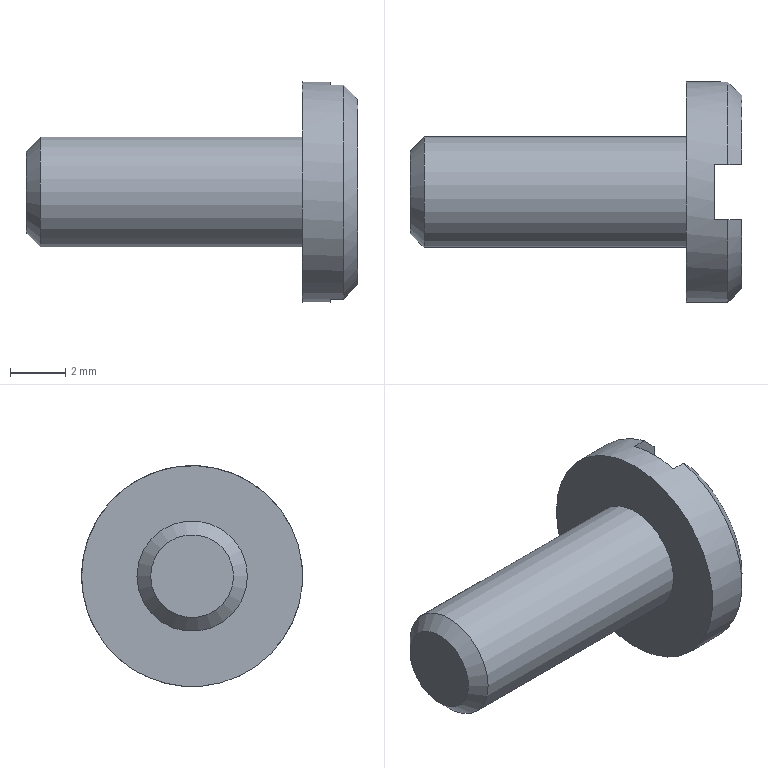Component | NX | SCREW | 1 solid | 12 faces | box 12 x 8 x 8 mm | volume 206 mm3 | plane 7 | cone 3 | cylinder 2 | commonest cylinder face diameters 4 x1 8 x1
STEP:
#1=CARTESIAN_POINT('',(0.,0.,0.));
#2=DIRECTION('',(0.,0.,1.));
#3=DIRECTION('',(1.,0.,0.));
#4=AXIS2_PLACEMENT_3D('',#1,#2,#3);
#5=CARTESIAN_POINT('',(63.511,118.396,33.354));
#6=VERTEX_POINT('',#5);
#7=CARTESIAN_POINT('',(63.511,118.396,26.646));
#8=VERTEX_POINT('',#7);
#9=CARTESIAN_POINT('',(63.511,118.396,35.5));
#10=DIRECTION('',(0.,0.,-1.));
#11=VECTOR('',#10,1.);
#12=LINE('',#9,#11);
#13=CARTESIAN_POINT('',(63.511,119.396,30.));
#14=DIRECTION('',(1.,0.,0.));
#15=DIRECTION('',(0.,1.,0.));
#16=AXIS2_PLACEMENT_3D('',#13,#14,#15);
#17=PLANE('',#16);
#18=CARTESIAN_POINT('',(-1.,5.5));
#19=DIRECTION('',(0.,-1.));
#20=VECTOR('',#19,1.);
#21=LINE('',#18,#20);
#22=(GEOMETRIC_REPRESENTATION_CONTEXT(2)PARAMETRIC_REPRESENTATION_CONTEXT()REPRESENTATION_CONTEXT('',''));
#23=DEFINITIONAL_REPRESENTATION('',(#21),#22);
#24=PCURVE('',#17,#23);
#25=CARTESIAN_POINT('',(62.511,118.396,35.5));
#26=DIRECTION('',(0.,-1.,-0.));
#27=DIRECTION('',(0.,0.,-1.));
#28=AXIS2_PLACEMENT_3D('',#25,#26,#27);
#29=PLANE('',#28);
#30=CARTESIAN_POINT('',(0.,1.));
#31=DIRECTION('',(1.,0.));
#32=VECTOR('',#31,1.);
#33=LINE('',#30,#32);
#34=(GEOMETRIC_REPRESENTATION_CONTEXT(2)PARAMETRIC_REPRESENTATION_CONTEXT()REPRESENTATION_CONTEXT('',''));
#35=DEFINITIONAL_REPRESENTATION('',(#33),#34);
#36=PCURVE('',#29,#35);
#37=SURFACE_CURVE('',#12,(#24,#36),.PCURVE_S1.);
#38=EDGE_CURVE('',#6,#8,#37,.T.);
#39=ORIENTED_EDGE('',*,*,#38,.F.);
#40=CARTESIAN_POINT('',(63.511,119.396,30.));
#41=DIRECTION('',(1.,0.,0.));
#42=DIRECTION('',(0.,1.,0.));
#43=AXIS2_PLACEMENT_3D('',#40,#41,#42);
#44=CIRCLE('',#43,3.5);
#45=CARTESIAN_POINT('',(0.,0.));
#46=DIRECTION('',(1.,0.));
#47=AXIS2_PLACEMENT_2D('',#45,#46);
#48=CIRCLE('',#47,3.5);
#49=(GEOMETRIC_REPRESENTATION_CONTEXT(2)PARAMETRIC_REPRESENTATION_CONTEXT()REPRESENTATION_CONTEXT('',''));
#50=DEFINITIONAL_REPRESENTATION('',(#48),#49);
#51=PCURVE('',#17,#50);
#52=CARTESIAN_POINT('',(63.511,119.396,30.));
#53=DIRECTION('',(-1.,0.,0.));
#54=DIRECTION('',(0.,-1.,0.));
#55=AXIS2_PLACEMENT_3D('',#52,#53,#54);
#56=CONICAL_SURFACE('',#55,3.5,0.7854);
#57=CARTESIAN_POINT('',(9.425,0.));
#58=DIRECTION('',(-1.,0.));
#59=VECTOR('',#58,1.);
#60=LINE('',#57,#59);
#61=(GEOMETRIC_REPRESENTATION_CONTEXT(2)PARAMETRIC_REPRESENTATION_CONTEXT()REPRESENTATION_CONTEXT('',''));
#62=DEFINITIONAL_REPRESENTATION('',(#60),#61);
#63=PCURVE('',#56,#62);
#64=SURFACE_CURVE('',#44,(#51,#63),.PCURVE_S1.);
#65=EDGE_CURVE('',#6,#8,#64,.T.);
#66=ORIENTED_EDGE('',*,*,#65,.T.);
#67=EDGE_LOOP('',(#39,#66));
#68=FACE_BOUND('',#67,.T.);
#69=ADVANCED_FACE('',(#68),#17,.T.);
#70=CARTESIAN_POINT('',(52.011,121.396,30.));
#71=VERTEX_POINT('',#70);
#72=CARTESIAN_POINT('',(52.011,119.396,30.));
#73=DIRECTION('',(1.,0.,0.));
#74=DIRECTION('',(0.,1.,0.));
#75=AXIS2_PLACEMENT_3D('',#72,#73,#74);
#76=CIRCLE('',#75,2.);
#77=CARTESIAN_POINT('',(61.511,119.396,30.));
#78=DIRECTION('',(-1.,0.,0.));
#79=DIRECTION('',(0.,-1.,0.));
#80=AXIS2_PLACEMENT_3D('',#77,#78,#79);
#81=CYLINDRICAL_SURFACE('',#80,2.);
#82=CARTESIAN_POINT('',(9.425,9.5));
#83=DIRECTION('',(-1.,0.));
#84=VECTOR('',#83,1.);
#85=LINE('',#82,#84);
#86=(GEOMETRIC_REPRESENTATION_CONTEXT(2)PARAMETRIC_REPRESENTATION_CONTEXT()REPRESENTATION_CONTEXT('',''));
#87=DEFINITIONAL_REPRESENTATION('',(#85),#86);
#88=PCURVE('',#81,#87);
#89=CARTESIAN_POINT('',(52.011,119.396,30.));
#90=DIRECTION('',(1.,0.,0.));
#91=DIRECTION('',(0.,1.,0.));
#92=AXIS2_PLACEMENT_3D('',#89,#90,#91);
#93=CONICAL_SURFACE('',#92,2.,0.7854);
#94=CARTESIAN_POINT('',(0.,0.));
#95=DIRECTION('',(1.,0.));
#96=VECTOR('',#95,1.);
#97=LINE('',#94,#96);
#98=(GEOMETRIC_REPRESENTATION_CONTEXT(2)PARAMETRIC_REPRESENTATION_CONTEXT()REPRESENTATION_CONTEXT('',''));
#99=DEFINITIONAL_REPRESENTATION('',(#97),#98);
#100=PCURVE('',#93,#99);
#101=SURFACE_CURVE('',#76,(#88,#100),.PCURVE_S1.);
#102=EDGE_CURVE('',#71,#71,#101,.T.);
#103=ORIENTED_EDGE('',*,*,#102,.T.);
#104=CARTESIAN_POINT('',(61.511,121.396,30.));
#105=VERTEX_POINT('',#104);
#106=CARTESIAN_POINT('',(61.511,121.396,30.));
#107=CARTESIAN_POINT('',(52.011,121.396,30.));
#108=B_SPLINE_CURVE_WITH_KNOTS('',1,(#106,#107),.UNSPECIFIED.,.F.,.F.,(2,2),(0.,9.5),.PIECEWISE_BEZIER_KNOTS.);
#109=CARTESIAN_POINT('',(3.142,0.));
#110=DIRECTION('',(0.,1.));
#111=VECTOR('',#110,1.);
#112=LINE('',#109,#111);
#113=(GEOMETRIC_REPRESENTATION_CONTEXT(2)PARAMETRIC_REPRESENTATION_CONTEXT()REPRESENTATION_CONTEXT('',''));
#114=DEFINITIONAL_REPRESENTATION('',(#112),#113);
#115=PCURVE('',#81,#114);
#116=CARTESIAN_POINT('',(9.425,0.));
#117=DIRECTION('',(0.,1.));
#118=VECTOR('',#117,1.);
#119=LINE('',#116,#118);
#120=(GEOMETRIC_REPRESENTATION_CONTEXT(2)PARAMETRIC_REPRESENTATION_CONTEXT()REPRESENTATION_CONTEXT('',''));
#121=DEFINITIONAL_REPRESENTATION('',(#119),#120);
#122=PCURVE('',#81,#121);
#123=SEAM_CURVE('',#108,(#115,#122),.PCURVE_S1.);
#124=EDGE_CURVE('',#105,#71,#123,.T.);
#125=ORIENTED_EDGE('',*,*,#124,.F.);
#126=CARTESIAN_POINT('',(61.511,119.396,30.));
#127=DIRECTION('',(1.,0.,0.));
#128=DIRECTION('',(0.,1.,0.));
#129=AXIS2_PLACEMENT_3D('',#126,#127,#128);
#130=CIRCLE('',#129,2.);
#131=CARTESIAN_POINT('',(9.425,0.));
#132=DIRECTION('',(-1.,0.));
#133=VECTOR('',#132,1.);
#134=LINE('',#131,#133);
#135=(GEOMETRIC_REPRESENTATION_CONTEXT(2)PARAMETRIC_REPRESENTATION_CONTEXT()REPRESENTATION_CONTEXT('',''));
#136=DEFINITIONAL_REPRESENTATION('',(#134),#135);
#137=PCURVE('',#81,#136);
#138=CARTESIAN_POINT('',(61.511,119.396,30.));
#139=DIRECTION('',(1.,0.,0.));
#140=DIRECTION('',(0.,1.,0.));
#141=AXIS2_PLACEMENT_3D('',#138,#139,#140);
#142=PLANE('',#141);
#143=CARTESIAN_POINT('',(0.,0.));
#144=DIRECTION('',(1.,0.));
#145=AXIS2_PLACEMENT_2D('',#143,#144);
#146=CIRCLE('',#145,2.);
#147=(GEOMETRIC_REPRESENTATION_CONTEXT(2)PARAMETRIC_REPRESENTATION_CONTEXT()REPRESENTATION_CONTEXT('',''));
#148=DEFINITIONAL_REPRESENTATION('',(#146),#147);
#149=PCURVE('',#142,#148);
#150=SURFACE_CURVE('',#130,(#137,#149),.PCURVE_S1.);
#151=EDGE_CURVE('',#105,#105,#150,.T.);
#152=ORIENTED_EDGE('',*,*,#151,.F.);
#153=ORIENTED_EDGE('',*,*,#124,.T.);
#154=EDGE_LOOP('',(#103,#125,#152,#153));
#155=FACE_BOUND('',#154,.T.);
#156=ADVANCED_FACE('',(#155),#81,.T.);
#157=CARTESIAN_POINT('',(51.511,120.896,30.));
#158=VERTEX_POINT('',#157);
#159=CARTESIAN_POINT('',(51.511,119.396,30.));
#160=DIRECTION('',(-1.,0.,0.));
#161=DIRECTION('',(0.,1.,0.));
#162=AXIS2_PLACEMENT_3D('',#159,#160,#161);
#163=CIRCLE('',#162,1.5);
#164=CARTESIAN_POINT('',(51.511,119.396,30.));
#165=DIRECTION('',(1.,0.,0.));
#166=DIRECTION('',(0.,1.,0.));
#167=AXIS2_PLACEMENT_3D('',#164,#165,#166);
#168=PLANE('',#167);
#169=CARTESIAN_POINT('',(1.5,0.));
#170=CARTESIAN_POINT('',(1.5,-2.598));
#171=CARTESIAN_POINT('',(-0.75,-1.299));
#172=CARTESIAN_POINT('',(-3.,-0.));
#173=CARTESIAN_POINT('',(-0.75,1.299));
#174=CARTESIAN_POINT('',(1.5,2.598));
#175=CARTESIAN_POINT('',(1.5,0.));
#176=(BOUNDED_CURVE()B_SPLINE_CURVE(2,(#169,#170,#171,#172,#173,#174,#175),.UNSPECIFIED.,.T.,.F.)B_SPLINE_CURVE_WITH_KNOTS((1,2,2,2,2,1),(-2.094,0.,2.094,4.189,6.283,8.378),.UNSPECIFIED.)CURVE()GEOMETRIC_REPRESENTATION_ITEM()RATIONAL_B_SPLINE_CURVE((1.,0.5,1.,0.5,1.,0.5,1.))REPRESENTATION_ITEM(''));
#177=(GEOMETRIC_REPRESENTATION_CONTEXT(2)PARAMETRIC_REPRESENTATION_CONTEXT()REPRESENTATION_CONTEXT('',''));
#178=DEFINITIONAL_REPRESENTATION('',(#176),#177);
#179=PCURVE('',#168,#178);
#180=CARTESIAN_POINT('',(6.283,-0.5));
#181=DIRECTION('',(-1.,0.));
#182=VECTOR('',#181,1.);
#183=LINE('',#180,#182);
#184=(GEOMETRIC_REPRESENTATION_CONTEXT(2)PARAMETRIC_REPRESENTATION_CONTEXT()REPRESENTATION_CONTEXT('',''));
#185=DEFINITIONAL_REPRESENTATION('',(#183),#184);
#186=PCURVE('',#93,#185);
#187=SURFACE_CURVE('',#163,(#179,#186),.PCURVE_S1.);
#188=EDGE_CURVE('',#158,#158,#187,.T.);
#189=ORIENTED_EDGE('',*,*,#188,.T.);
#190=EDGE_LOOP('',(#189));
#191=FACE_BOUND('',#190,.T.);
#192=ADVANCED_FACE('',(#191),#168,.F.);
#193=CARTESIAN_POINT('',(62.511,118.396,26.127));
#194=VERTEX_POINT('',#193);
#195=CARTESIAN_POINT('',(63.011,118.396,26.127));
#196=VERTEX_POINT('',#195);
#197=CARTESIAN_POINT('',(63.511,118.396,26.127));
#198=DIRECTION('',(1.,0.,0.));
#199=VECTOR('',#198,1.);
#200=LINE('',#197,#199);
#201=CARTESIAN_POINT('',(63.511,119.396,30.));
#202=DIRECTION('',(-1.,0.,0.));
#203=DIRECTION('',(0.,-1.,0.));
#204=AXIS2_PLACEMENT_3D('',#201,#202,#203);
#205=CYLINDRICAL_SURFACE('',#204,4.);
#206=CARTESIAN_POINT('',(4.965,0.));
#207=DIRECTION('',(0.,-1.));
#208=VECTOR('',#207,1.);
#209=LINE('',#206,#208);
#210=(GEOMETRIC_REPRESENTATION_CONTEXT(2)PARAMETRIC_REPRESENTATION_CONTEXT()REPRESENTATION_CONTEXT('',''));
#211=DEFINITIONAL_REPRESENTATION('',(#209),#210);
#212=PCURVE('',#205,#211);
#213=CARTESIAN_POINT('',(9.373,1.));
#214=DIRECTION('',(0.,1.));
#215=VECTOR('',#214,1.);
#216=LINE('',#213,#215);
#217=(GEOMETRIC_REPRESENTATION_CONTEXT(2)PARAMETRIC_REPRESENTATION_CONTEXT()REPRESENTATION_CONTEXT('',''));
#218=DEFINITIONAL_REPRESENTATION('',(#216),#217);
#219=PCURVE('',#29,#218);
#220=SURFACE_CURVE('',#200,(#212,#219),.PCURVE_S1.);
#221=EDGE_CURVE('',#194,#196,#220,.T.);
#222=ORIENTED_EDGE('',*,*,#221,.T.);
#223=CARTESIAN_POINT('',(63.011,118.396,33.873));
#224=VERTEX_POINT('',#223);
#225=CARTESIAN_POINT('',(63.011,119.396,30.));
#226=DIRECTION('',(-1.,0.,0.));
#227=DIRECTION('',(0.,1.,0.));
#228=AXIS2_PLACEMENT_3D('',#225,#226,#227);
#229=CIRCLE('',#228,4.);
#230=CARTESIAN_POINT('',(3.142,0.5));
#231=DIRECTION('',(1.,0.));
#232=VECTOR('',#231,1.);
#233=LINE('',#230,#232);
#234=(GEOMETRIC_REPRESENTATION_CONTEXT(2)PARAMETRIC_REPRESENTATION_CONTEXT()REPRESENTATION_CONTEXT('',''));
#235=DEFINITIONAL_REPRESENTATION('',(#233),#234);
#236=PCURVE('',#205,#235);
#237=CARTESIAN_POINT('',(3.142,0.5));
#238=DIRECTION('',(1.,-0.));
#239=VECTOR('',#238,1.);
#240=LINE('',#237,#239);
#241=(GEOMETRIC_REPRESENTATION_CONTEXT(2)PARAMETRIC_REPRESENTATION_CONTEXT()REPRESENTATION_CONTEXT('',''));
#242=DEFINITIONAL_REPRESENTATION('',(#240),#241);
#243=PCURVE('',#56,#242);
#244=SURFACE_CURVE('',#229,(#236,#243),.PCURVE_S1.);
#245=EDGE_CURVE('',#196,#224,#244,.T.);
#246=ORIENTED_EDGE('',*,*,#245,.T.);
#247=CARTESIAN_POINT('',(62.511,118.396,33.873));
#248=VERTEX_POINT('',#247);
#249=CARTESIAN_POINT('',(63.511,118.396,33.873));
#250=DIRECTION('',(-1.,0.,0.));
#251=VECTOR('',#250,1.);
#252=LINE('',#249,#251);
#253=CARTESIAN_POINT('',(7.601,0.));
#254=DIRECTION('',(0.,1.));
#255=VECTOR('',#254,1.);
#256=LINE('',#253,#255);
#257=(GEOMETRIC_REPRESENTATION_CONTEXT(2)PARAMETRIC_REPRESENTATION_CONTEXT()REPRESENTATION_CONTEXT('',''));
#258=DEFINITIONAL_REPRESENTATION('',(#256),#257);
#259=PCURVE('',#205,#258);
#260=CARTESIAN_POINT('',(1.627,1.));
#261=DIRECTION('',(0.,-1.));
#262=VECTOR('',#261,1.);
#263=LINE('',#260,#262);
#264=(GEOMETRIC_REPRESENTATION_CONTEXT(2)PARAMETRIC_REPRESENTATION_CONTEXT()REPRESENTATION_CONTEXT('',''));
#265=DEFINITIONAL_REPRESENTATION('',(#263),#264);
#266=PCURVE('',#29,#265);
#267=SURFACE_CURVE('',#252,(#259,#266),.PCURVE_S1.);
#268=EDGE_CURVE('',#224,#248,#267,.T.);
#269=ORIENTED_EDGE('',*,*,#268,.T.);
#270=CARTESIAN_POINT('',(62.511,120.396,33.873));
#271=VERTEX_POINT('',#270);
#272=CARTESIAN_POINT('',(62.511,119.396,30.));
#273=DIRECTION('',(1.,0.,0.));
#274=DIRECTION('',(0.,1.,0.));
#275=AXIS2_PLACEMENT_3D('',#272,#273,#274);
#276=CIRCLE('',#275,4.);
#277=CARTESIAN_POINT('',(9.425,1.));
#278=DIRECTION('',(-1.,0.));
#279=VECTOR('',#278,1.);
#280=LINE('',#277,#279);
#281=(GEOMETRIC_REPRESENTATION_CONTEXT(2)PARAMETRIC_REPRESENTATION_CONTEXT()REPRESENTATION_CONTEXT('',''));
#282=DEFINITIONAL_REPRESENTATION('',(#280),#281);
#283=PCURVE('',#205,#282);
#284=CARTESIAN_POINT('',(62.511,119.396,30.));
#285=DIRECTION('',(1.,0.,0.));
#286=DIRECTION('',(0.,1.,0.));
#287=AXIS2_PLACEMENT_3D('',#284,#285,#286);
#288=PLANE('',#287);
#289=CARTESIAN_POINT('',(0.,0.));
#290=DIRECTION('',(1.,0.));
#291=AXIS2_PLACEMENT_2D('',#289,#290);
#292=CIRCLE('',#291,4.);
#293=(GEOMETRIC_REPRESENTATION_CONTEXT(2)PARAMETRIC_REPRESENTATION_CONTEXT()REPRESENTATION_CONTEXT('',''));
#294=DEFINITIONAL_REPRESENTATION('',(#292),#293);
#295=PCURVE('',#288,#294);
#296=SURFACE_CURVE('',#276,(#283,#295),.PCURVE_S1.);
#297=EDGE_CURVE('',#271,#248,#296,.T.);
#298=ORIENTED_EDGE('',*,*,#297,.F.);
#299=CARTESIAN_POINT('',(63.011,120.396,33.873));
#300=VERTEX_POINT('',#299);
#301=CARTESIAN_POINT('',(63.511,120.396,33.873));
#302=DIRECTION('',(1.,0.,0.));
#303=VECTOR('',#302,1.);
#304=LINE('',#301,#303);
#305=CARTESIAN_POINT('',(8.107,0.));
#306=DIRECTION('',(0.,-1.));
#307=VECTOR('',#306,1.);
#308=LINE('',#305,#307);
#309=(GEOMETRIC_REPRESENTATION_CONTEXT(2)PARAMETRIC_REPRESENTATION_CONTEXT()REPRESENTATION_CONTEXT('',''));
#310=DEFINITIONAL_REPRESENTATION('',(#308),#309);
#311=PCURVE('',#205,#310);
#312=CARTESIAN_POINT('',(62.511,120.396,25.));
#313=DIRECTION('',(0.,1.,0.));
#314=DIRECTION('',(0.,-0.,1.));
#315=AXIS2_PLACEMENT_3D('',#312,#313,#314);
#316=PLANE('',#315);
#317=CARTESIAN_POINT('',(8.873,1.));
#318=DIRECTION('',(0.,1.));
#319=VECTOR('',#318,1.);
#320=LINE('',#317,#319);
#321=(GEOMETRIC_REPRESENTATION_CONTEXT(2)PARAMETRIC_REPRESENTATION_CONTEXT()REPRESENTATION_CONTEXT('',''));
#322=DEFINITIONAL_REPRESENTATION('',(#320),#321);
#323=PCURVE('',#316,#322);
#324=SURFACE_CURVE('',#304,(#311,#323),.PCURVE_S1.);
#325=EDGE_CURVE('',#271,#300,#324,.T.);
#326=ORIENTED_EDGE('',*,*,#325,.T.);
#327=CARTESIAN_POINT('',(63.011,120.396,26.127));
#328=VERTEX_POINT('',#327);
#329=CARTESIAN_POINT('',(63.011,119.396,30.));
#330=DIRECTION('',(-1.,0.,0.));
#331=DIRECTION('',(0.,1.,0.));
#332=AXIS2_PLACEMENT_3D('',#329,#330,#331);
#333=CIRCLE('',#332,4.);
#334=CARTESIAN_POINT('',(3.142,0.5));
#335=DIRECTION('',(1.,0.));
#336=VECTOR('',#335,1.);
#337=LINE('',#334,#336);
#338=(GEOMETRIC_REPRESENTATION_CONTEXT(2)PARAMETRIC_REPRESENTATION_CONTEXT()REPRESENTATION_CONTEXT('',''));
#339=DEFINITIONAL_REPRESENTATION('',(#337),#338);
#340=PCURVE('',#205,#339);
#341=CARTESIAN_POINT('',(63.511,119.396,30.));
#342=DIRECTION('',(-1.,0.,0.));
#343=DIRECTION('',(0.,-1.,0.));
#344=AXIS2_PLACEMENT_3D('',#341,#342,#343);
#345=CONICAL_SURFACE('',#344,3.5,0.7854);
#346=CARTESIAN_POINT('',(-3.142,0.5));
#347=DIRECTION('',(1.,-0.));
#348=VECTOR('',#347,1.);
#349=LINE('',#346,#348);
#350=(GEOMETRIC_REPRESENTATION_CONTEXT(2)PARAMETRIC_REPRESENTATION_CONTEXT()REPRESENTATION_CONTEXT('',''));
#351=DEFINITIONAL_REPRESENTATION('',(#349),#350);
#352=PCURVE('',#345,#351);
#353=SURFACE_CURVE('',#333,(#340,#352),.PCURVE_S1.);
#354=EDGE_CURVE('',#300,#328,#353,.T.);
#355=ORIENTED_EDGE('',*,*,#354,.T.);
#356=CARTESIAN_POINT('',(62.511,120.396,26.127));
#357=VERTEX_POINT('',#356);
#358=CARTESIAN_POINT('',(63.511,120.396,26.127));
#359=DIRECTION('',(-1.,0.,0.));
#360=VECTOR('',#359,1.);
#361=LINE('',#358,#360);
#362=CARTESIAN_POINT('',(10.743,0.));
#363=DIRECTION('',(0.,1.));
#364=VECTOR('',#363,1.);
#365=LINE('',#362,#364);
#366=(GEOMETRIC_REPRESENTATION_CONTEXT(2)PARAMETRIC_REPRESENTATION_CONTEXT()REPRESENTATION_CONTEXT('',''));
#367=DEFINITIONAL_REPRESENTATION('',(#365),#366);
#368=PCURVE('',#205,#367);
#369=CARTESIAN_POINT('',(1.127,1.));
#370=DIRECTION('',(0.,-1.));
#371=VECTOR('',#370,1.);
#372=LINE('',#369,#371);
#373=(GEOMETRIC_REPRESENTATION_CONTEXT(2)PARAMETRIC_REPRESENTATION_CONTEXT()REPRESENTATION_CONTEXT('',''));
#374=DEFINITIONAL_REPRESENTATION('',(#372),#373);
#375=PCURVE('',#316,#374);
#376=SURFACE_CURVE('',#361,(#368,#375),.PCURVE_S1.);
#377=EDGE_CURVE('',#328,#357,#376,.T.);
#378=ORIENTED_EDGE('',*,*,#377,.T.);
#379=CARTESIAN_POINT('',(62.511,119.396,30.));
#380=DIRECTION('',(1.,0.,0.));
#381=DIRECTION('',(0.,1.,0.));
#382=AXIS2_PLACEMENT_3D('',#379,#380,#381);
#383=CIRCLE('',#382,4.);
#384=CARTESIAN_POINT('',(15.708,1.));
#385=DIRECTION('',(-1.,0.));
#386=VECTOR('',#385,1.);
#387=LINE('',#384,#386);
#388=(GEOMETRIC_REPRESENTATION_CONTEXT(2)PARAMETRIC_REPRESENTATION_CONTEXT()REPRESENTATION_CONTEXT('',''));
#389=DEFINITIONAL_REPRESENTATION('',(#387),#388);
#390=PCURVE('',#205,#389);
#391=CARTESIAN_POINT('',(0.,0.));
#392=DIRECTION('',(1.,0.));
#393=AXIS2_PLACEMENT_2D('',#391,#392);
#394=CIRCLE('',#393,4.);
#395=(GEOMETRIC_REPRESENTATION_CONTEXT(2)PARAMETRIC_REPRESENTATION_CONTEXT()REPRESENTATION_CONTEXT('',''));
#396=DEFINITIONAL_REPRESENTATION('',(#394),#395);
#397=PCURVE('',#288,#396);
#398=SURFACE_CURVE('',#383,(#390,#397),.PCURVE_S1.);
#399=EDGE_CURVE('',#194,#357,#398,.T.);
#400=ORIENTED_EDGE('',*,*,#399,.F.);
#401=CARTESIAN_POINT('',(61.511,118.396,26.127));
#402=VERTEX_POINT('',#401);
#403=CARTESIAN_POINT('',(62.511,118.396,26.127));
#404=CARTESIAN_POINT('',(61.511,118.396,26.127));
#405=B_SPLINE_CURVE_WITH_KNOTS('',1,(#403,#404),.UNSPECIFIED.,.F.,.F.,(2,2),(1.,2.),.PIECEWISE_BEZIER_KNOTS.);
#406=CARTESIAN_POINT('',(11.248,0.));
#407=DIRECTION('',(0.,1.));
#408=VECTOR('',#407,1.);
#409=LINE('',#406,#408);
#410=(GEOMETRIC_REPRESENTATION_CONTEXT(2)PARAMETRIC_REPRESENTATION_CONTEXT()REPRESENTATION_CONTEXT('',''));
#411=DEFINITIONAL_REPRESENTATION('',(#409),#410);
#412=PCURVE('',#205,#411);
#413=CARTESIAN_POINT('',(4.965,0.));
#414=DIRECTION('',(0.,1.));
#415=VECTOR('',#414,1.);
#416=LINE('',#413,#415);
#417=(GEOMETRIC_REPRESENTATION_CONTEXT(2)PARAMETRIC_REPRESENTATION_CONTEXT()REPRESENTATION_CONTEXT('',''));
#418=DEFINITIONAL_REPRESENTATION('',(#416),#417);
#419=PCURVE('',#205,#418);
#420=SEAM_CURVE('',#405,(#412,#419),.PCURVE_S1.);
#421=EDGE_CURVE('',#194,#402,#420,.T.);
#422=ORIENTED_EDGE('',*,*,#421,.T.);
#423=CARTESIAN_POINT('',(61.511,123.396,30.));
#424=VERTEX_POINT('',#423);
#425=CARTESIAN_POINT('',(61.511,119.396,30.));
#426=DIRECTION('',(1.,0.,0.));
#427=DIRECTION('',(0.,1.,0.));
#428=AXIS2_PLACEMENT_3D('',#425,#426,#427);
#429=CIRCLE('',#428,4.);
#430=CARTESIAN_POINT('',(15.708,2.));
#431=DIRECTION('',(-1.,0.));
#432=VECTOR('',#431,1.);
#433=LINE('',#430,#432);
#434=(GEOMETRIC_REPRESENTATION_CONTEXT(2)PARAMETRIC_REPRESENTATION_CONTEXT()REPRESENTATION_CONTEXT('',''));
#435=DEFINITIONAL_REPRESENTATION('',(#433),#434);
#436=PCURVE('',#205,#435);
#437=CARTESIAN_POINT('',(0.,0.));
#438=DIRECTION('',(1.,0.));
#439=AXIS2_PLACEMENT_2D('',#437,#438);
#440=CIRCLE('',#439,4.);
#441=(GEOMETRIC_REPRESENTATION_CONTEXT(2)PARAMETRIC_REPRESENTATION_CONTEXT()REPRESENTATION_CONTEXT('',''));
#442=DEFINITIONAL_REPRESENTATION('',(#440),#441);
#443=PCURVE('',#142,#442);
#444=SURFACE_CURVE('',#429,(#436,#443),.PCURVE_S1.);
#445=EDGE_CURVE('',#402,#424,#444,.T.);
#446=ORIENTED_EDGE('',*,*,#445,.T.);
#447=CARTESIAN_POINT('',(61.511,119.396,30.));
#448=DIRECTION('',(1.,0.,0.));
#449=DIRECTION('',(0.,1.,0.));
#450=AXIS2_PLACEMENT_3D('',#447,#448,#449);
#451=CIRCLE('',#450,4.);
#452=CARTESIAN_POINT('',(9.425,2.));
#453=DIRECTION('',(-1.,0.));
#454=VECTOR('',#453,1.);
#455=LINE('',#452,#454);
#456=(GEOMETRIC_REPRESENTATION_CONTEXT(2)PARAMETRIC_REPRESENTATION_CONTEXT()REPRESENTATION_CONTEXT('',''));
#457=DEFINITIONAL_REPRESENTATION('',(#455),#456);
#458=PCURVE('',#205,#457);
#459=CARTESIAN_POINT('',(0.,0.));
#460=DIRECTION('',(1.,0.));
#461=AXIS2_PLACEMENT_2D('',#459,#460);
#462=CIRCLE('',#461,4.);
#463=(GEOMETRIC_REPRESENTATION_CONTEXT(2)PARAMETRIC_REPRESENTATION_CONTEXT()REPRESENTATION_CONTEXT('',''));
#464=DEFINITIONAL_REPRESENTATION('',(#462),#463);
#465=PCURVE('',#142,#464);
#466=SURFACE_CURVE('',#451,(#458,#465),.PCURVE_S1.);
#467=EDGE_CURVE('',#424,#402,#466,.T.);
#468=ORIENTED_EDGE('',*,*,#467,.T.);
#469=ORIENTED_EDGE('',*,*,#421,.F.);
#470=EDGE_LOOP('',(#222,#246,#269,#298,#326,#355,#378,#400,#422,#446,#468,#469));
#471=FACE_BOUND('',#470,.T.);
#472=ADVANCED_FACE('',(#471),#205,.T.);
#473=CARTESIAN_POINT('',(63.511,120.396,26.646));
#474=VERTEX_POINT('',#473);
#475=CARTESIAN_POINT('',(63.511,120.396,33.354));
#476=VERTEX_POINT('',#475);
#477=CARTESIAN_POINT('',(63.511,120.396,25.));
#478=DIRECTION('',(0.,-0.,1.));
#479=VECTOR('',#478,1.);
#480=LINE('',#477,#479);
#481=CARTESIAN_POINT('',(63.511,119.396,30.));
#482=DIRECTION('',(1.,0.,0.));
#483=DIRECTION('',(0.,1.,0.));
#484=AXIS2_PLACEMENT_3D('',#481,#482,#483);
#485=PLANE('',#484);
#486=CARTESIAN_POINT('',(1.,-5.));
#487=DIRECTION('',(-0.,1.));
#488=VECTOR('',#487,1.);
#489=LINE('',#486,#488);
#490=(GEOMETRIC_REPRESENTATION_CONTEXT(2)PARAMETRIC_REPRESENTATION_CONTEXT()REPRESENTATION_CONTEXT('',''));
#491=DEFINITIONAL_REPRESENTATION('',(#489),#490);
#492=PCURVE('',#485,#491);
#493=CARTESIAN_POINT('',(0.,1.));
#494=DIRECTION('',(1.,0.));
#495=VECTOR('',#494,1.);
#496=LINE('',#493,#495);
#497=(GEOMETRIC_REPRESENTATION_CONTEXT(2)PARAMETRIC_REPRESENTATION_CONTEXT()REPRESENTATION_CONTEXT('',''));
#498=DEFINITIONAL_REPRESENTATION('',(#496),#497);
#499=PCURVE('',#316,#498);
#500=SURFACE_CURVE('',#480,(#492,#499),.PCURVE_S1.);
#501=EDGE_CURVE('',#474,#476,#500,.T.);
#502=ORIENTED_EDGE('',*,*,#501,.F.);
#503=CARTESIAN_POINT('',(63.511,119.396,30.));
#504=DIRECTION('',(1.,0.,0.));
#505=DIRECTION('',(0.,1.,0.));
#506=AXIS2_PLACEMENT_3D('',#503,#504,#505);
#507=CIRCLE('',#506,3.5);
#508=CARTESIAN_POINT('',(0.,0.));
#509=DIRECTION('',(1.,0.));
#510=AXIS2_PLACEMENT_2D('',#508,#509);
#511=CIRCLE('',#510,3.5);
#512=(GEOMETRIC_REPRESENTATION_CONTEXT(2)PARAMETRIC_REPRESENTATION_CONTEXT()REPRESENTATION_CONTEXT('',''));
#513=DEFINITIONAL_REPRESENTATION('',(#511),#512);
#514=PCURVE('',#485,#513);
#515=CARTESIAN_POINT('',(9.425,0.));
#516=DIRECTION('',(-1.,0.));
#517=VECTOR('',#516,1.);
#518=LINE('',#515,#517);
#519=(GEOMETRIC_REPRESENTATION_CONTEXT(2)PARAMETRIC_REPRESENTATION_CONTEXT()REPRESENTATION_CONTEXT('',''));
#520=DEFINITIONAL_REPRESENTATION('',(#518),#519);
#521=PCURVE('',#345,#520);
#522=SURFACE_CURVE('',#507,(#514,#521),.PCURVE_S1.);
#523=EDGE_CURVE('',#474,#476,#522,.T.);
#524=ORIENTED_EDGE('',*,*,#523,.T.);
#525=EDGE_LOOP('',(#502,#524));
#526=FACE_BOUND('',#525,.T.);
#527=ADVANCED_FACE('',(#526),#485,.T.);
#528=ORIENTED_EDGE('',*,*,#151,.T.);
#529=EDGE_LOOP('',(#528));
#530=FACE_BOUND('',#529,.T.);
#531=ORIENTED_EDGE('',*,*,#467,.F.);
#532=ORIENTED_EDGE('',*,*,#445,.F.);
#533=EDGE_LOOP('',(#531,#532));
#534=FACE_BOUND('',#533,.T.);
#535=ADVANCED_FACE('',(#530,#534),#142,.F.);
#536=ORIENTED_EDGE('',*,*,#297,.T.);
#537=CARTESIAN_POINT('',(62.511,118.396,35.5));
#538=DIRECTION('',(0.,-0.,1.));
#539=VECTOR('',#538,1.);
#540=LINE('',#537,#539);
#541=CARTESIAN_POINT('',(-1.,5.5));
#542=DIRECTION('',(-0.,1.));
#543=VECTOR('',#542,1.);
#544=LINE('',#541,#543);
#545=(GEOMETRIC_REPRESENTATION_CONTEXT(2)PARAMETRIC_REPRESENTATION_CONTEXT()REPRESENTATION_CONTEXT('',''));
#546=DEFINITIONAL_REPRESENTATION('',(#544),#545);
#547=PCURVE('',#288,#546);
#548=CARTESIAN_POINT('',(0.,0.));
#549=DIRECTION('',(-1.,0.));
#550=VECTOR('',#549,1.);
#551=LINE('',#548,#550);
#552=(GEOMETRIC_REPRESENTATION_CONTEXT(2)PARAMETRIC_REPRESENTATION_CONTEXT()REPRESENTATION_CONTEXT('',''));
#553=DEFINITIONAL_REPRESENTATION('',(#551),#552);
#554=PCURVE('',#29,#553);
#555=SURFACE_CURVE('',#540,(#547,#554),.PCURVE_S1.);
#556=EDGE_CURVE('',#194,#248,#555,.T.);
#557=ORIENTED_EDGE('',*,*,#556,.F.);
#558=ORIENTED_EDGE('',*,*,#399,.T.);
#559=CARTESIAN_POINT('',(62.511,120.396,25.));
#560=DIRECTION('',(0.,0.,-1.));
#561=VECTOR('',#560,1.);
#562=LINE('',#559,#561);
#563=CARTESIAN_POINT('',(1.,-5.));
#564=DIRECTION('',(0.,-1.));
#565=VECTOR('',#564,1.);
#566=LINE('',#563,#565);
#567=(GEOMETRIC_REPRESENTATION_CONTEXT(2)PARAMETRIC_REPRESENTATION_CONTEXT()REPRESENTATION_CONTEXT('',''));
#568=DEFINITIONAL_REPRESENTATION('',(#566),#567);
#569=PCURVE('',#288,#568);
#570=CARTESIAN_POINT('',(0.,0.));
#571=DIRECTION('',(-1.,0.));
#572=VECTOR('',#571,1.);
#573=LINE('',#570,#572);
#574=(GEOMETRIC_REPRESENTATION_CONTEXT(2)PARAMETRIC_REPRESENTATION_CONTEXT()REPRESENTATION_CONTEXT('',''));
#575=DEFINITIONAL_REPRESENTATION('',(#573),#574);
#576=PCURVE('',#316,#575);
#577=SURFACE_CURVE('',#562,(#569,#576),.PCURVE_S1.);
#578=EDGE_CURVE('',#271,#357,#577,.T.);
#579=ORIENTED_EDGE('',*,*,#578,.F.);
#580=EDGE_LOOP('',(#536,#557,#558,#579));
#581=FACE_BOUND('',#580,.T.);
#582=ADVANCED_FACE('',(#581),#288,.T.);
#583=ORIENTED_EDGE('',*,*,#38,.T.);
#584=CARTESIAN_POINT('',(63.511,118.396,26.646));
#585=CARTESIAN_POINT('',(63.344,118.396,26.472));
#586=CARTESIAN_POINT('',(63.178,118.396,26.3));
#587=CARTESIAN_POINT('',(63.011,118.396,26.127));
#588=B_SPLINE_CURVE_WITH_KNOTS('',3,(#584,#585,#586,#587),.UNSPECIFIED.,.F.,.F.,(4,4),(0.,1.),.PIECEWISE_BEZIER_KNOTS.);
#589=CARTESIAN_POINT('',(8.854,1.));
#590=CARTESIAN_POINT('',(9.028,0.8338));
#591=CARTESIAN_POINT('',(9.2,0.6671));
#592=CARTESIAN_POINT('',(9.373,0.5));
#593=B_SPLINE_CURVE_WITH_KNOTS('',3,(#589,#590,#591,#592),.UNSPECIFIED.,.F.,.F.,(4,4),(0.,1.),.PIECEWISE_BEZIER_KNOTS.);
#594=(GEOMETRIC_REPRESENTATION_CONTEXT(2)PARAMETRIC_REPRESENTATION_CONTEXT()REPRESENTATION_CONTEXT('',''));
#595=DEFINITIONAL_REPRESENTATION('',(#593),#594);
#596=PCURVE('',#29,#595);
#597=CARTESIAN_POINT('',(5.002,0.));
#598=CARTESIAN_POINT('',(4.965,0.5));
#599=B_SPLINE_CURVE_WITH_KNOTS('',1,(#597,#598),.UNSPECIFIED.,.F.,.F.,(2,2),(0.,1.),.PIECEWISE_BEZIER_KNOTS.);
#600=(GEOMETRIC_REPRESENTATION_CONTEXT(2)PARAMETRIC_REPRESENTATION_CONTEXT()REPRESENTATION_CONTEXT('',''));
#601=DEFINITIONAL_REPRESENTATION('',(#599),#600);
#602=PCURVE('',#56,#601);
#603=SURFACE_CURVE('',#588,(#596,#602),.PCURVE_S1.);
#604=EDGE_CURVE('',#8,#196,#603,.T.);
#605=ORIENTED_EDGE('',*,*,#604,.T.);
#606=ORIENTED_EDGE('',*,*,#221,.F.);
#607=ORIENTED_EDGE('',*,*,#556,.T.);
#608=ORIENTED_EDGE('',*,*,#268,.F.);
#609=CARTESIAN_POINT('',(63.011,118.396,33.873));
#610=CARTESIAN_POINT('',(63.178,118.396,33.7));
#611=CARTESIAN_POINT('',(63.344,118.396,33.528));
#612=CARTESIAN_POINT('',(63.511,118.396,33.354));
#613=B_SPLINE_CURVE_WITH_KNOTS('',3,(#609,#610,#611,#612),.UNSPECIFIED.,.F.,.F.,(4,4),(0.,1.),.PIECEWISE_BEZIER_KNOTS.);
#614=CARTESIAN_POINT('',(1.627,0.5));
#615=CARTESIAN_POINT('',(1.8,0.6671));
#616=CARTESIAN_POINT('',(1.972,0.8338));
#617=CARTESIAN_POINT('',(2.146,1.));
#618=B_SPLINE_CURVE_WITH_KNOTS('',3,(#614,#615,#616,#617),.UNSPECIFIED.,.F.,.F.,(4,4),(0.,1.),.PIECEWISE_BEZIER_KNOTS.);
#619=(GEOMETRIC_REPRESENTATION_CONTEXT(2)PARAMETRIC_REPRESENTATION_CONTEXT()REPRESENTATION_CONTEXT('',''));
#620=DEFINITIONAL_REPRESENTATION('',(#618),#619);
#621=PCURVE('',#29,#620);
#622=CARTESIAN_POINT('',(7.601,0.5));
#623=CARTESIAN_POINT('',(7.564,0.));
#624=B_SPLINE_CURVE_WITH_KNOTS('',1,(#622,#623),.UNSPECIFIED.,.F.,.F.,(2,2),(0.,1.),.PIECEWISE_BEZIER_KNOTS.);
#625=(GEOMETRIC_REPRESENTATION_CONTEXT(2)PARAMETRIC_REPRESENTATION_CONTEXT()REPRESENTATION_CONTEXT('',''));
#626=DEFINITIONAL_REPRESENTATION('',(#624),#625);
#627=PCURVE('',#56,#626);
#628=SURFACE_CURVE('',#613,(#621,#627),.PCURVE_S1.);
#629=EDGE_CURVE('',#224,#6,#628,.T.);
#630=ORIENTED_EDGE('',*,*,#629,.T.);
#631=EDGE_LOOP('',(#583,#605,#606,#607,#608,#630));
#632=FACE_BOUND('',#631,.T.);
#633=ADVANCED_FACE('',(#632),#29,.F.);
#634=ORIENTED_EDGE('',*,*,#501,.T.);
#635=CARTESIAN_POINT('',(63.511,120.396,33.354));
#636=CARTESIAN_POINT('',(63.344,120.396,33.528));
#637=CARTESIAN_POINT('',(63.178,120.396,33.7));
#638=CARTESIAN_POINT('',(63.011,120.396,33.873));
#639=B_SPLINE_CURVE_WITH_KNOTS('',3,(#635,#636,#637,#638),.UNSPECIFIED.,.F.,.F.,(4,4),(0.,1.),.PIECEWISE_BEZIER_KNOTS.);
#640=CARTESIAN_POINT('',(8.354,1.));
#641=CARTESIAN_POINT('',(8.528,0.8338));
#642=CARTESIAN_POINT('',(8.7,0.6671));
#643=CARTESIAN_POINT('',(8.873,0.5));
#644=B_SPLINE_CURVE_WITH_KNOTS('',3,(#640,#641,#642,#643),.UNSPECIFIED.,.F.,.F.,(4,4),(0.,1.),.PIECEWISE_BEZIER_KNOTS.);
#645=(GEOMETRIC_REPRESENTATION_CONTEXT(2)PARAMETRIC_REPRESENTATION_CONTEXT()REPRESENTATION_CONTEXT('',''));
#646=DEFINITIONAL_REPRESENTATION('',(#644),#645);
#647=PCURVE('',#316,#646);
#648=CARTESIAN_POINT('',(1.861,0.));
#649=CARTESIAN_POINT('',(1.823,0.5));
#650=B_SPLINE_CURVE_WITH_KNOTS('',1,(#648,#649),.UNSPECIFIED.,.F.,.F.,(2,2),(0.,1.),.PIECEWISE_BEZIER_KNOTS.);
#651=(GEOMETRIC_REPRESENTATION_CONTEXT(2)PARAMETRIC_REPRESENTATION_CONTEXT()REPRESENTATION_CONTEXT('',''));
#652=DEFINITIONAL_REPRESENTATION('',(#650),#651);
#653=PCURVE('',#345,#652);
#654=SURFACE_CURVE('',#639,(#647,#653),.PCURVE_S1.);
#655=EDGE_CURVE('',#476,#300,#654,.T.);
#656=ORIENTED_EDGE('',*,*,#655,.T.);
#657=ORIENTED_EDGE('',*,*,#325,.F.);
#658=ORIENTED_EDGE('',*,*,#578,.T.);
#659=ORIENTED_EDGE('',*,*,#377,.F.);
#660=CARTESIAN_POINT('',(63.011,120.396,26.127));
#661=CARTESIAN_POINT('',(63.178,120.396,26.3));
#662=CARTESIAN_POINT('',(63.344,120.396,26.472));
#663=CARTESIAN_POINT('',(63.511,120.396,26.646));
#664=B_SPLINE_CURVE_WITH_KNOTS('',3,(#660,#661,#662,#663),.UNSPECIFIED.,.F.,.F.,(4,4),(0.,1.),.PIECEWISE_BEZIER_KNOTS.);
#665=CARTESIAN_POINT('',(1.127,0.5));
#666=CARTESIAN_POINT('',(1.3,0.6671));
#667=CARTESIAN_POINT('',(1.472,0.8338));
#668=CARTESIAN_POINT('',(1.646,1.));
#669=B_SPLINE_CURVE_WITH_KNOTS('',3,(#665,#666,#667,#668),.UNSPECIFIED.,.F.,.F.,(4,4),(0.,1.),.PIECEWISE_BEZIER_KNOTS.);
#670=(GEOMETRIC_REPRESENTATION_CONTEXT(2)PARAMETRIC_REPRESENTATION_CONTEXT()REPRESENTATION_CONTEXT('',''));
#671=DEFINITIONAL_REPRESENTATION('',(#669),#670);
#672=PCURVE('',#316,#671);
#673=CARTESIAN_POINT('',(4.46,0.5));
#674=CARTESIAN_POINT('',(4.423,0.));
#675=B_SPLINE_CURVE_WITH_KNOTS('',1,(#673,#674),.UNSPECIFIED.,.F.,.F.,(2,2),(0.,1.),.PIECEWISE_BEZIER_KNOTS.);
#676=(GEOMETRIC_REPRESENTATION_CONTEXT(2)PARAMETRIC_REPRESENTATION_CONTEXT()REPRESENTATION_CONTEXT('',''));
#677=DEFINITIONAL_REPRESENTATION('',(#675),#676);
#678=PCURVE('',#345,#677);
#679=SURFACE_CURVE('',#664,(#672,#678),.PCURVE_S1.);
#680=EDGE_CURVE('',#328,#474,#679,.T.);
#681=ORIENTED_EDGE('',*,*,#680,.T.);
#682=EDGE_LOOP('',(#634,#656,#657,#658,#659,#681));
#683=FACE_BOUND('',#682,.T.);
#684=ADVANCED_FACE('',(#683),#316,.F.);
#685=ORIENTED_EDGE('',*,*,#188,.F.);
#686=CARTESIAN_POINT('',(51.511,120.896,30.));
#687=CARTESIAN_POINT('',(52.011,121.396,30.));
#688=B_SPLINE_CURVE_WITH_KNOTS('',1,(#686,#687),.UNSPECIFIED.,.F.,.F.,(2,2),(-0.7071,0.),.PIECEWISE_BEZIER_KNOTS.);
#689=CARTESIAN_POINT('',(6.283,0.));
#690=DIRECTION('',(0.,1.));
#691=VECTOR('',#690,1.);
#692=LINE('',#689,#691);
#693=(GEOMETRIC_REPRESENTATION_CONTEXT(2)PARAMETRIC_REPRESENTATION_CONTEXT()REPRESENTATION_CONTEXT('',''));
#694=DEFINITIONAL_REPRESENTATION('',(#692),#693);
#695=PCURVE('',#93,#694);
#696=CARTESIAN_POINT('',(0.,0.));
#697=DIRECTION('',(0.,1.));
#698=VECTOR('',#697,1.);
#699=LINE('',#696,#698);
#700=(GEOMETRIC_REPRESENTATION_CONTEXT(2)PARAMETRIC_REPRESENTATION_CONTEXT()REPRESENTATION_CONTEXT('',''));
#701=DEFINITIONAL_REPRESENTATION('',(#699),#700);
#702=PCURVE('',#93,#701);
#703=SEAM_CURVE('',#688,(#695,#702),.PCURVE_S1.);
#704=EDGE_CURVE('',#158,#71,#703,.T.);
#705=ORIENTED_EDGE('',*,*,#704,.T.);
#706=ORIENTED_EDGE('',*,*,#102,.F.);
#707=ORIENTED_EDGE('',*,*,#704,.F.);
#708=EDGE_LOOP('',(#685,#705,#706,#707));
#709=FACE_BOUND('',#708,.T.);
#710=ADVANCED_FACE('',(#709),#93,.T.);
#711=ORIENTED_EDGE('',*,*,#629,.F.);
#712=ORIENTED_EDGE('',*,*,#245,.F.);
#713=ORIENTED_EDGE('',*,*,#604,.F.);
#714=ORIENTED_EDGE('',*,*,#65,.F.);
#715=EDGE_LOOP('',(#711,#712,#713,#714));
#716=FACE_BOUND('',#715,.T.);
#717=ADVANCED_FACE('',(#716),#56,.T.);
#718=ORIENTED_EDGE('',*,*,#680,.F.);
#719=ORIENTED_EDGE('',*,*,#354,.F.);
#720=ORIENTED_EDGE('',*,*,#655,.F.);
#721=ORIENTED_EDGE('',*,*,#523,.F.);
#722=EDGE_LOOP('',(#718,#719,#720,#721));
#723=FACE_BOUND('',#722,.T.);
#724=ADVANCED_FACE('',(#723),#345,.T.);
#725=CLOSED_SHELL('',(#69,#156,#192,#472,#527,#535,#582,#633,#684,#710,#717,#724));
#726=MANIFOLD_SOLID_BREP('',#725);
#727=(LENGTH_UNIT()NAMED_UNIT(*)SI_UNIT(.MILLI.,.METRE.));
#728=UNCERTAINTY_MEASURE_WITH_UNIT(LENGTH_MEASURE(0.002),#727,'','');
#729=(NAMED_UNIT(*)PLANE_ANGLE_UNIT()SI_UNIT($,.RADIAN.));
#730=(NAMED_UNIT(*)SI_UNIT($,.STERADIAN.)SOLID_ANGLE_UNIT());
#731=(GEOMETRIC_REPRESENTATION_CONTEXT(3)GLOBAL_UNCERTAINTY_ASSIGNED_CONTEXT((#728))GLOBAL_UNIT_ASSIGNED_CONTEXT((#727,#729,#730))REPRESENTATION_CONTEXT('',''));
#732=ADVANCED_BREP_SHAPE_REPRESENTATION('',(#4,#726),#731);